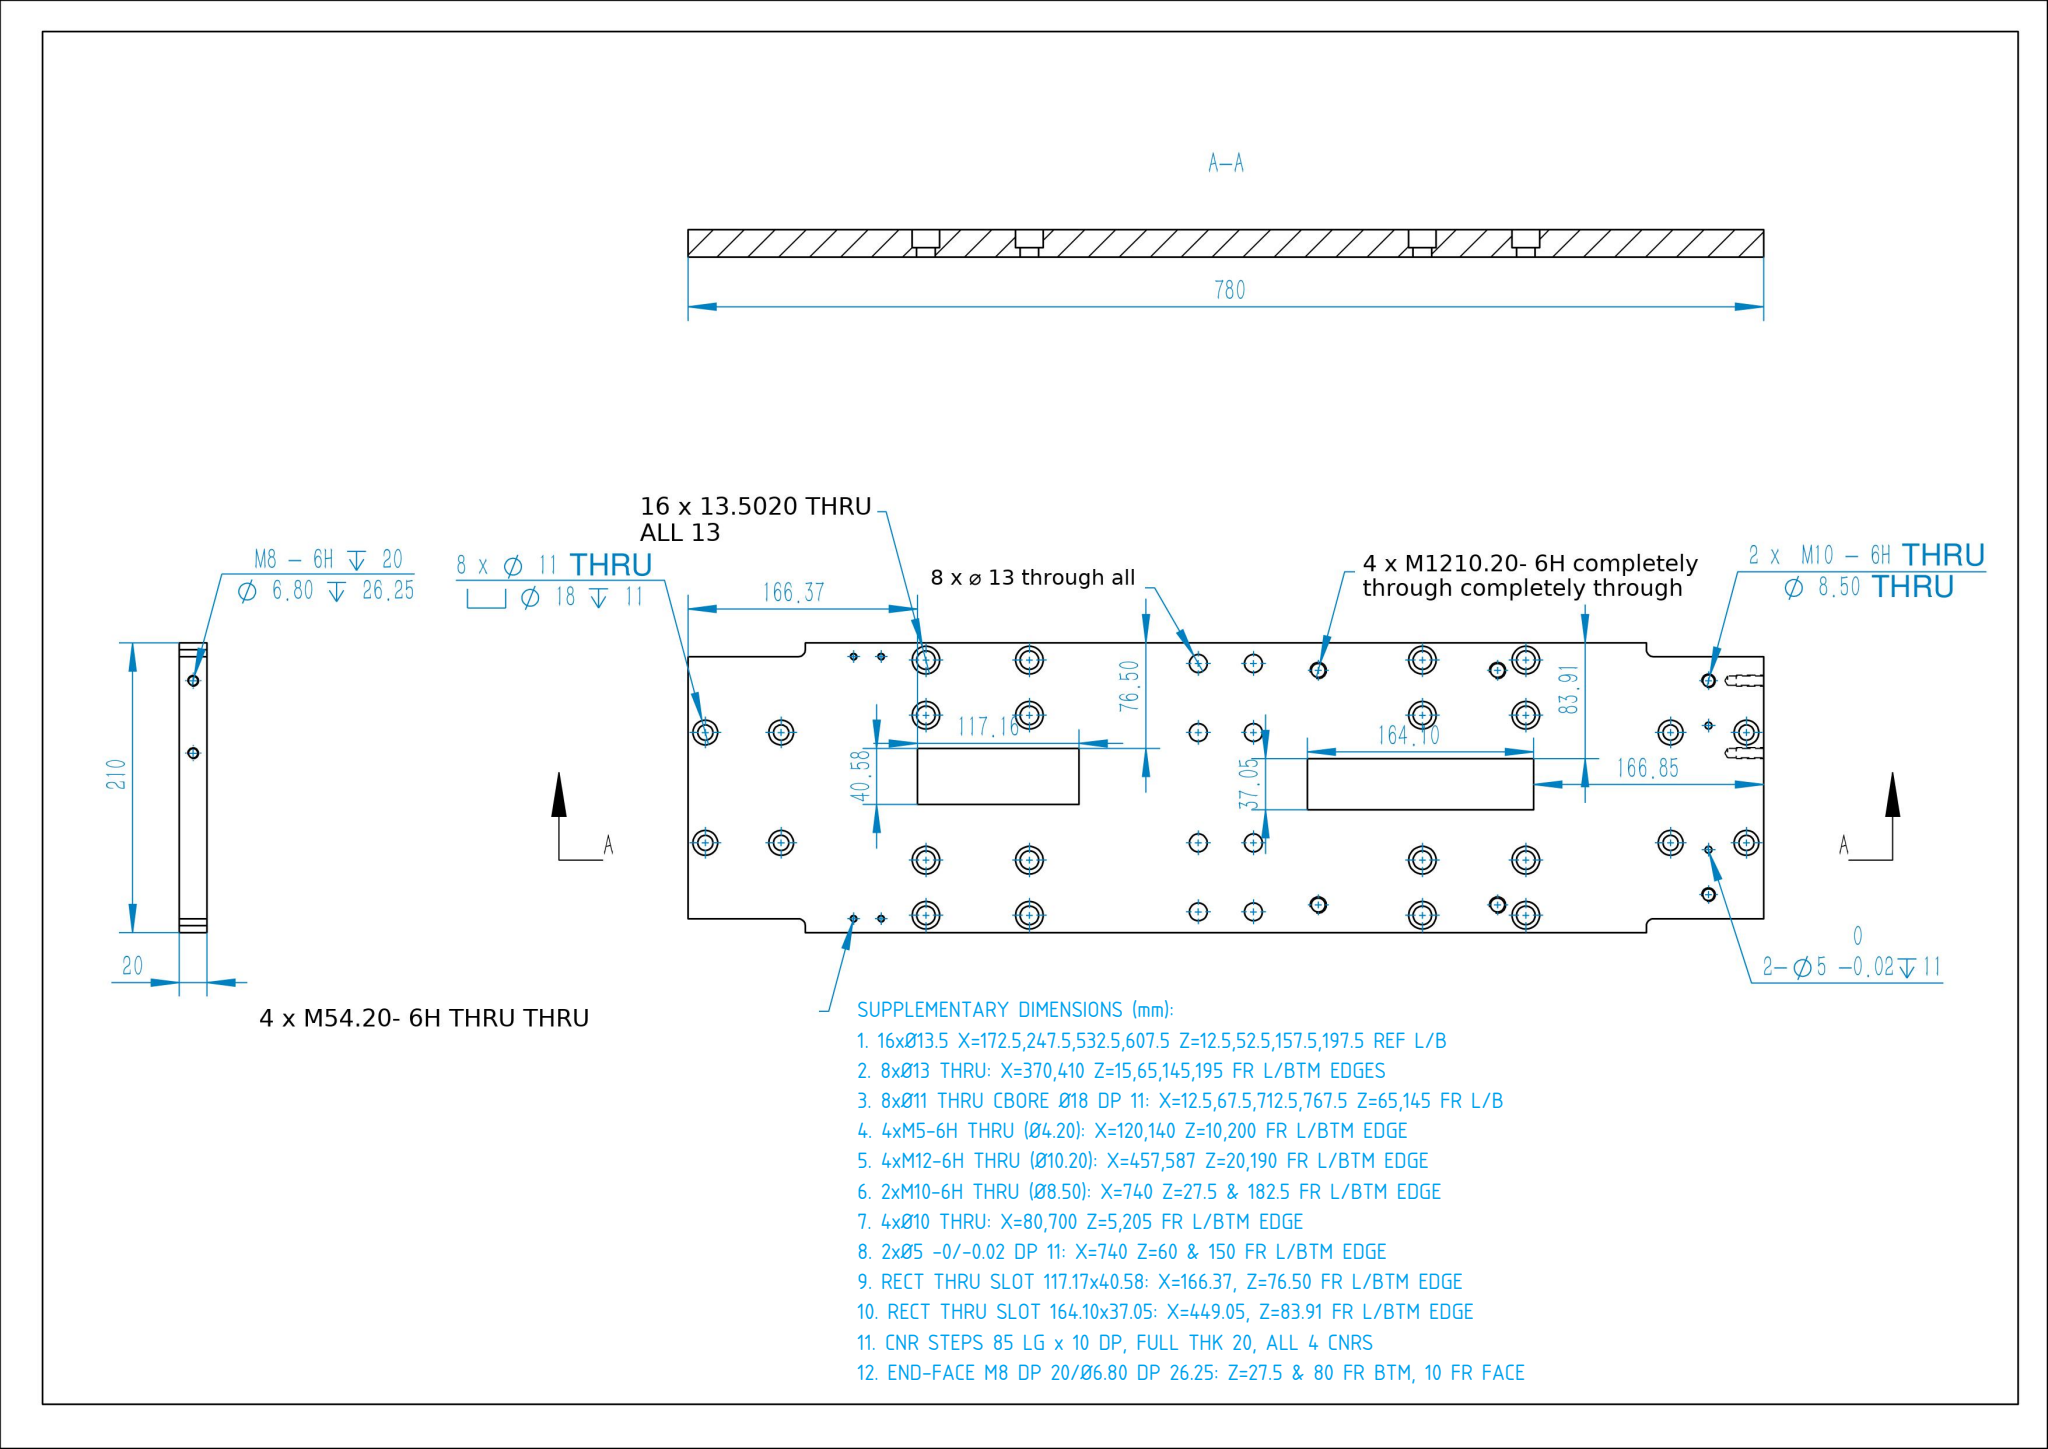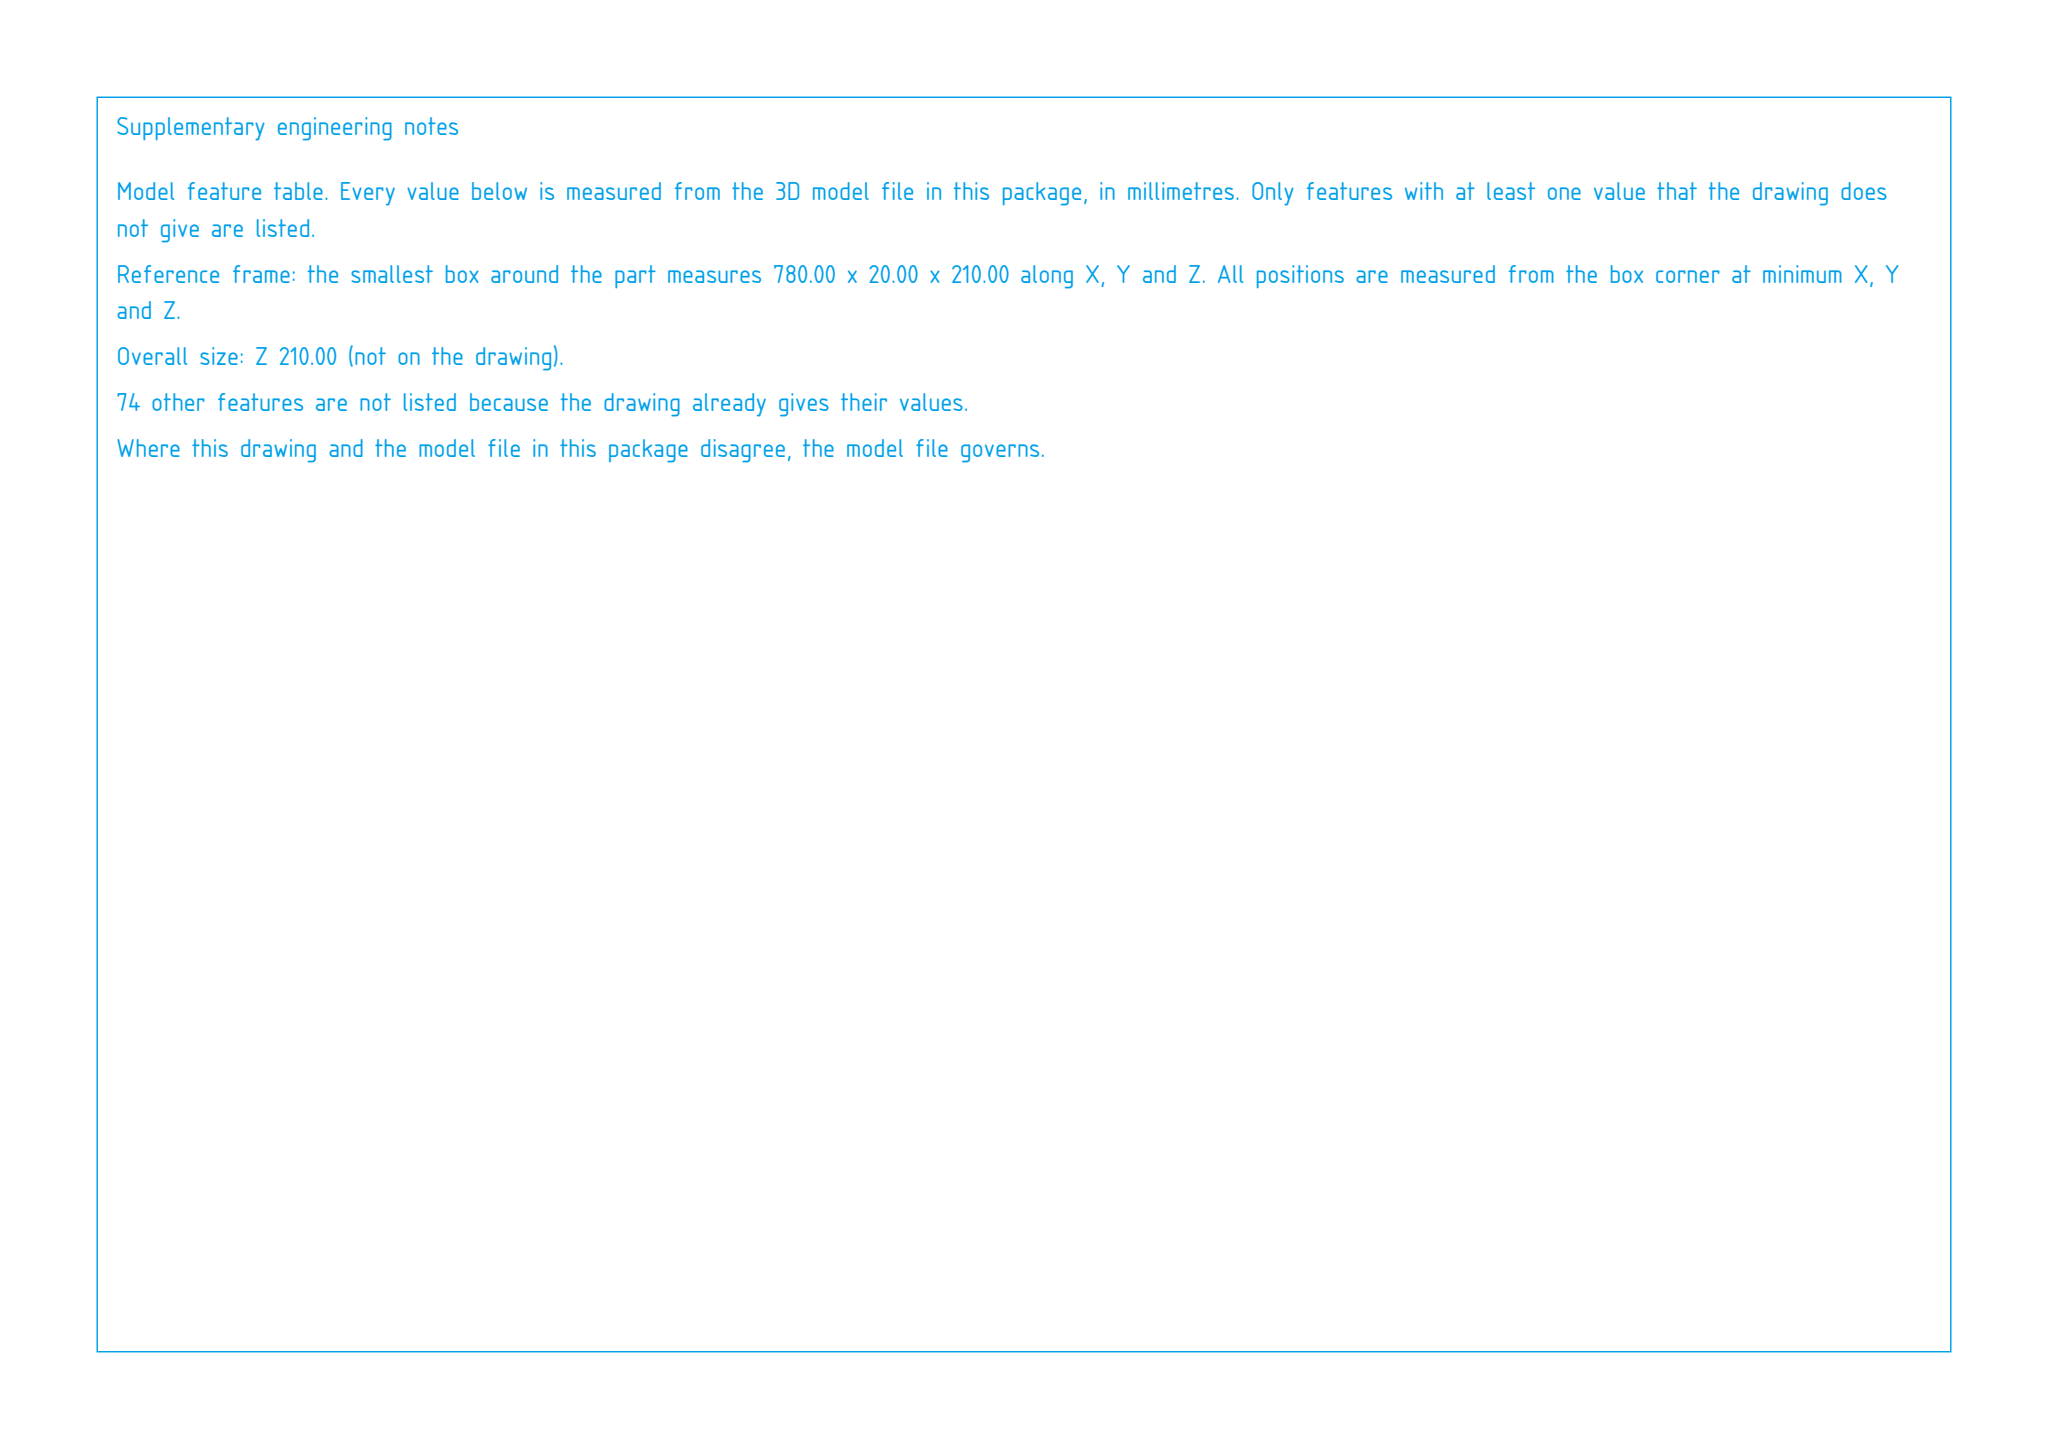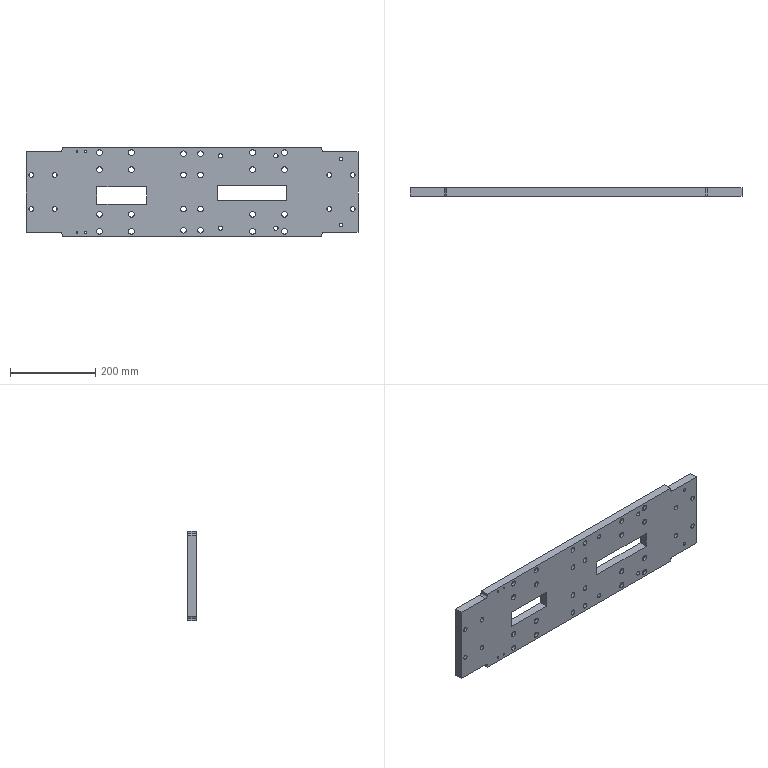Part | SolidWorks | mm | 1 solid | 196 faces | box 780 x 20 x 210 mm | volume 2847563 mm3 | cylinder 144 | plane 48 | cone 4 | commonest cylinder face diameters 20 x32 13.5 x32 13 x16 18 x16 11 x16 4.2 x8 10.2 x8 6.8 x4
build123d program:
from build123d import *

# Parameters (mm, degrees)
SKETCH1_W                                         = 780
SKETCH1_H                                         = 210
BOSS_EXTRUDE1_DEPTH                               = 10
SKETCH2_W                                         = 85
SKETCH2_H                                         = 10
CUT_EXTRUDE1_DEPTH                                = 405.382
FILLET1_R                                         = 5
HOLE_SIZE_ACCORDING_TO_HEXAGON_SOCKET_D           = 11
HOLE_SIZE_ACCORDING_TO_HEXAGON_SOCKET_CBORE_D     = 18
HOLE_SIZE_ACCORDING_TO_HEXAGON_SOCKET_CBORE_DEPTH = 11
HOLE_SIZE_ACCORDING_TO_HEXAGON_SOC_2_D            = 13.5
HOLE_SIZE_ACCORDING_TO_HEXAGON_SOC_2_CBORE_D      = 20
HOLE_SIZE_ACCORDING_TO_HEXAGON_SOC_2_CBORE_DEPTH  = 13
F_13_0_13_DIAMETER_HOLE2_D                        = 13
M10_TAPPED_HOLE1_D                                = 8.5
SKETCH13_R                                        = 2.5
CUT_EXTRUDE2_DEPTH                                = 11
M12_TAPPED_HOLE1_D                                = 10.2
M8_TAPPED_HOLE1_D                                 = 6.8
M8_TAPPED_HOLE1_DEPTH                             = 26.25
M8_TAPPED_HOLE1_TIP                               = 2.043
M8_TAPPED_HOLE2_D                                 = 6.8
M8_TAPPED_HOLE2_DEPTH                             = 26.25
M8_TAPPED_HOLE2_TIP                               = 2.043
M5_TAPPED_HOLE1_D                                 = 4.2
SKETCH22_W                                        = 117.164
SKETCH22_H                                        = 40.584
SKETCH22_W_2                                      = 164.1
SKETCH22_H_2                                      = 37.055
CUT_EXTRUDE3_DEPTH                                = 146


with BuildPart() as part:
    # Sketch1 → Boss-Extrude1 (new, symmetric)
    with BuildSketch(Plane(origin=(0, 0, 0), x_dir=(1, 0, 0), z_dir=(0, 1, 0))):
        Rectangle(SKETCH1_W, SKETCH1_H)
    extrude(amount=BOSS_EXTRUDE1_DEPTH, both=True)

    # Sketch2 → Cut-Extrude1 (cut, through all)
    with BuildSketch(Plane(origin=(0, 10, 0), x_dir=(1, 0, 0), z_dir=(0, 1, 0))):
        with Locations((-347.5, 100)):
            Rectangle(SKETCH2_W, SKETCH2_H)
        with Locations((347.5, 100)):
            Rectangle(SKETCH2_W, SKETCH2_H)
        with Locations((347.5, -100)):
            Rectangle(SKETCH2_W, SKETCH2_H)
        with Locations((-347.5, -100)):
            Rectangle(SKETCH2_W, SKETCH2_H)
    extrude(amount=-CUT_EXTRUDE1_DEPTH, mode=Mode.SUBTRACT)

    # Fillet1
    fillet1_edges = [part.edges().sort_by_distance(p)[0] for p in [
        (-305, 0, -95),
        (305, 0, -95),
        (305, 0, 95),
        (-305, 0, 95),
    ]]
    fillet(fillet1_edges, radius=FILLET1_R)

    # Hole Size _according to_ Hexagon Socket (through all)
    with Locations(Plane(origin=(0, 10, 0), x_dir=(1, 0, 0), z_dir=(0, 1, 0))):
        with Locations((-377.5, 40), (-322.5, 40), (-377.5, -40), (-322.5, -40), (322.5, -40), (377.5, -40), (322.5, 40), (377.5, 40)):
            CounterBoreHole(HOLE_SIZE_ACCORDING_TO_HEXAGON_SOCKET_D / 2, HOLE_SIZE_ACCORDING_TO_HEXAGON_SOCKET_CBORE_D / 2, HOLE_SIZE_ACCORDING_TO_HEXAGON_SOCKET_CBORE_DEPTH)

    # Hole Size _according to_ Hexagon Soc 2 (through all)
    with Locations(Plane(origin=(0, 10, 0), x_dir=(1, 0, 0), z_dir=(0, 1, 0))):
        with Locations((-217.5, -52.5), (-142.5, -52.5), (-217.5, -92.5), (-142.5, -92.5), (142.5, -92.5), (217.5, -92.5), (142.5, -52.5), (217.5, -52.5), (-142.5, 92.5), (-217.5, 92.5), (-142.5, 52.5), (-217.5, 52.5), (217.5, 52.5), (142.5, 52.5), (217.5, 92.5), (142.5, 92.5)):
            CounterBoreHole(HOLE_SIZE_ACCORDING_TO_HEXAGON_SOC_2_D / 2, HOLE_SIZE_ACCORDING_TO_HEXAGON_SOC_2_CBORE_D / 2, HOLE_SIZE_ACCORDING_TO_HEXAGON_SOC_2_CBORE_DEPTH)

    # 13.0 _13_ Diameter Hole2 (through all)
    with Locations(Plane(origin=(0, 10, 0), x_dir=(1, 0, 0), z_dir=(0, 1, 0))):
        with Locations((-20, 90), (-20, 40), (20, 90), (20, 40), (-20, -40), (-20, -90), (20, -40), (20, -90)):
            Hole(F_13_0_13_DIAMETER_HOLE2_D / 2)

    # M10 Tapped Hole1 (through all)
    with Locations(Plane(origin=(0, 10, 0), x_dir=(1, 0, 0), z_dir=(0, 1, 0))):
        with Locations((350, 77.5), (350, -77.5)):
            Hole(M10_TAPPED_HOLE1_D / 2)

    # Sketch13 → Cut-Extrude2 (cut)
    with BuildSketch(Plane(origin=(0, 10, 0), x_dir=(1, 0, 0), z_dir=(0, 1, 0))):
        with Locations(Location((350, -45, 0), (0, 0, 270))):
            Circle(SKETCH13_R)
        with Locations(Location((350, 45, 0), (0, 0, 90))):
            Circle(SKETCH13_R)
    extrude(amount=-CUT_EXTRUDE2_DEPTH, mode=Mode.SUBTRACT)

    # M12 Tapped Hole1 (through all)
    with Locations(Plane(origin=(0, 10, 0), x_dir=(1, 0, 0), z_dir=(0, 1, 0))):
        with Locations((197, 85), (67, 85), (67, -85), (197, -85)):
            Hole(M12_TAPPED_HOLE1_D / 2)

    # M8 Tapped Hole1
    with Locations(Plane(origin=(390, 0, 0), x_dir=(0, 0, -1), z_dir=(1, 0, 0))):
        with Locations((25, 0)):
            Hole(M8_TAPPED_HOLE1_D / 2, depth=M8_TAPPED_HOLE1_DEPTH)
            with Locations((0, 0, -(M8_TAPPED_HOLE1_DEPTH + M8_TAPPED_HOLE1_TIP / 2))):  # 118° drill point
                Cone(0, M8_TAPPED_HOLE1_D / 2, M8_TAPPED_HOLE1_TIP, mode=Mode.SUBTRACT)

    # M8 Tapped Hole2
    with Locations(Plane(origin=(390, 0, 0), x_dir=(0, 0, -1), z_dir=(1, 0, 0))):
        with Locations((77.5, 0)):
            Hole(M8_TAPPED_HOLE2_D / 2, depth=M8_TAPPED_HOLE2_DEPTH)
            with Locations((0, 0, -(M8_TAPPED_HOLE2_DEPTH + M8_TAPPED_HOLE2_TIP / 2))):  # 118° drill point
                Cone(0, M8_TAPPED_HOLE2_D / 2, M8_TAPPED_HOLE2_TIP, mode=Mode.SUBTRACT)

    # M5 Tapped Hole1 (through all)
    with Locations(Plane(origin=(0, 10, 0), x_dir=(1, 0, 0), z_dir=(0, 1, 0))):
        with Locations((-270, -95), (-250, -95), (-250, 95), (-270, 95)):
            Hole(M5_TAPPED_HOLE1_D / 2)

    # Sketch22 → Cut-Extrude3 (cut)
    with BuildSketch(Plane(origin=(0, 10, 0), x_dir=(1, 0, 0), z_dir=(0, 1, 0))):
        with Locations((-165.047, 8.211)):
            Rectangle(SKETCH22_W, SKETCH22_H)
        with Locations((141.097, 2.565)):
            Rectangle(SKETCH22_W_2, SKETCH22_H_2)
    extrude(amount=-CUT_EXTRUDE3_DEPTH, mode=Mode.SUBTRACT)


solid = part.part